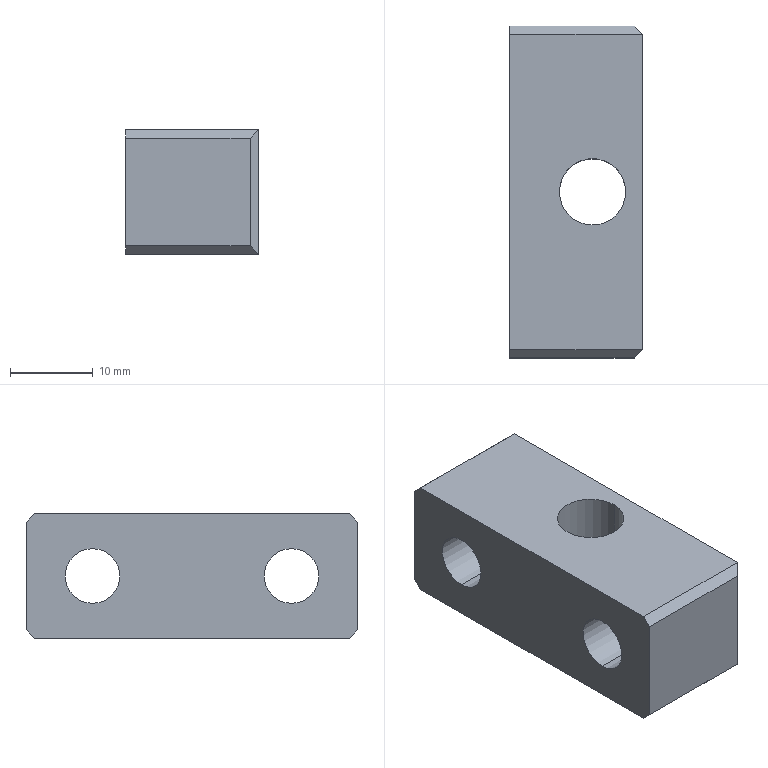Component | SolidWorks | ConveyorScrewAdjustmentSeat-2 | 1 solid | 24 faces | box 16 x 40 x 15 mm | volume 6635 mm3 | plane 14 | cylinder 10 | commonest cylinder face diameters 11 x4 6.6 x4 8 x2 | material Plain Carbon Steel
build123d program:
from build123d import *

# Parameters (mm, degrees)
SKETCH1_W                                            = 15
SKETCH1_H                                            = 40
BOSS_EXTRUDE1_DEPTH                                  = 16
HOLE_SIZE_ACCORDING_TO_TYPE_1_OF_HEXAGON_D           = 6.6
HOLE_SIZE_ACCORDING_TO_TYPE_1_OF_HEXAGON_CBORE_D     = 11
HOLE_SIZE_ACCORDING_TO_TYPE_1_OF_HEXAGON_CBORE_DEPTH = 8.8
M8_TAPPED_HOLE1_D                                    = 8
CHAMFER1_SIZE                                        = 1


with BuildPart() as part:
    # Sketch1 → Boss-Extrude1 (new body)
    with BuildSketch(Plane(origin=(0, 0, 0), x_dir=(0, 0, -1), z_dir=(1, 0, 0))):
        Rectangle(SKETCH1_W, SKETCH1_H)
    extrude(amount=BOSS_EXTRUDE1_DEPTH)

    # Hole Size according to type 1 of hexagon (through all)
    with Locations(Plane(origin=(16, 0, 0), x_dir=(0, 0, -1), z_dir=(1, 0, 0))):
        with Locations((0, 12), (0, -12)):
            CounterBoreHole(HOLE_SIZE_ACCORDING_TO_TYPE_1_OF_HEXAGON_D / 2, HOLE_SIZE_ACCORDING_TO_TYPE_1_OF_HEXAGON_CBORE_D / 2, HOLE_SIZE_ACCORDING_TO_TYPE_1_OF_HEXAGON_CBORE_DEPTH)

    # M8 Tapped Hole1 (through all)
    with Locations(Plane.XY.offset(7.5)):
        with Locations((10, 0)):
            Hole(M8_TAPPED_HOLE1_D / 2)

    # Chamfer1
    chamfer1_edges = [part.edges().sort_by_distance(p)[0] for p in [
        (16, -20, 0),
        (16, 20, 0),
        (8, -20, -7.5),
        (8, -20, 7.5),
        (8, 20, 7.5),
        (8, 20, -7.5),
    ]]
    chamfer(chamfer1_edges, length=CHAMFER1_SIZE)


solid = part.part

# Placed as in the assembly
solid = solid.moved(Location((47.45, 5.646, 262.5), (0, 0, 0)))
STEP:
#1=COLOUR_RGB('',0.7922,0.8196,0.9333);
#2=FILL_AREA_STYLE_COLOUR('',#1);
#3=FILL_AREA_STYLE('',(#2));
#4=SURFACE_STYLE_FILL_AREA(#3);
#5=SURFACE_SIDE_STYLE('',(#4));
#6=SURFACE_STYLE_USAGE(.BOTH.,#5);
#7=PRESENTATION_STYLE_ASSIGNMENT((#6));
#8=CARTESIAN_POINT('',(2.104,0.2223,10.039));
#9=VERTEX_POINT('',#8);
#10=CARTESIAN_POINT('',(2.419,0.2223,10.039));
#11=VERTEX_POINT('',#10);
#12=CARTESIAN_POINT('',(2.262,0.2223,10.039));
#13=DIRECTION('',(0.,0.,1.));
#14=DIRECTION('',(1.,0.,0.));
#15=AXIS2_PLACEMENT_3D('',#12,#13,#14);
#16=CIRCLE('',#15,0.1575);
#17=EDGE_CURVE('',#9,#11,#16,.T.);
#18=ORIENTED_EDGE('',*,*,#17,.F.);
#19=CARTESIAN_POINT('',(2.104,0.2223,10.63));
#20=VERTEX_POINT('',#19);
#21=CARTESIAN_POINT('',(2.104,0.2223,10.63));
#22=DIRECTION('',(0.,0.,1.));
#23=VECTOR('',#22,39.37);
#24=LINE('',#21,#23);
#25=EDGE_CURVE('',#9,#20,#24,.T.);
#26=ORIENTED_EDGE('',*,*,#25,.T.);
#27=CARTESIAN_POINT('',(2.419,0.2223,10.63));
#28=VERTEX_POINT('',#27);
#29=CARTESIAN_POINT('',(2.262,0.2223,10.63));
#30=DIRECTION('',(0.,0.,1.));
#31=DIRECTION('',(1.,0.,0.));
#32=AXIS2_PLACEMENT_3D('',#29,#30,#31);
#33=CIRCLE('',#32,0.1575);
#34=EDGE_CURVE('',#20,#28,#33,.T.);
#35=ORIENTED_EDGE('',*,*,#34,.T.);
#36=CARTESIAN_POINT('',(2.419,0.2223,10.63));
#37=DIRECTION('',(0.,0.,1.));
#38=VECTOR('',#37,39.37);
#39=LINE('',#36,#38);
#40=EDGE_CURVE('',#11,#28,#39,.T.);
#41=ORIENTED_EDGE('',*,*,#40,.F.);
#42=EDGE_LOOP('',(#18,#26,#35,#41));
#43=FACE_OUTER_BOUND('',#42,.T.);
#44=CARTESIAN_POINT('',(2.262,0.2223,10.63));
#45=DIRECTION('',(0.,0.,1.));
#46=DIRECTION('',(1.,0.,0.));
#47=AXIS2_PLACEMENT_3D('',#44,#45,#46);
#48=CYLINDRICAL_SURFACE('',#47,0.1575);
#49=ADVANCED_FACE('',(#43),#48,.F.);
#50=CARTESIAN_POINT('',(2.152,0.6947,10.551));
#51=VERTEX_POINT('',#50);
#52=CARTESIAN_POINT('',(2.152,0.6947,10.118));
#53=VERTEX_POINT('',#52);
#54=CARTESIAN_POINT('',(2.152,0.6947,10.335));
#55=DIRECTION('',(1.,0.,0.));
#56=DIRECTION('',(0.,0.,-1.));
#57=AXIS2_PLACEMENT_3D('',#54,#55,#56);
#58=CIRCLE('',#57,0.2165);
#59=EDGE_CURVE('',#51,#53,#58,.T.);
#60=ORIENTED_EDGE('',*,*,#59,.F.);
#61=CARTESIAN_POINT('',(2.498,0.6947,10.551));
#62=VERTEX_POINT('',#61);
#63=CARTESIAN_POINT('',(2.498,0.6947,10.551));
#64=DIRECTION('',(1.,0.,0.));
#65=VECTOR('',#64,39.37);
#66=LINE('',#63,#65);
#67=EDGE_CURVE('',#51,#62,#66,.T.);
#68=ORIENTED_EDGE('',*,*,#67,.T.);
#69=CARTESIAN_POINT('',(2.498,0.6947,10.118));
#70=VERTEX_POINT('',#69);
#71=CARTESIAN_POINT('',(2.498,0.6947,10.335));
#72=DIRECTION('',(1.,0.,0.));
#73=DIRECTION('',(0.,0.,-1.));
#74=AXIS2_PLACEMENT_3D('',#71,#72,#73);
#75=CIRCLE('',#74,0.2165);
#76=EDGE_CURVE('',#62,#70,#75,.T.);
#77=ORIENTED_EDGE('',*,*,#76,.T.);
#78=CARTESIAN_POINT('',(2.498,0.6947,10.118));
#79=DIRECTION('',(1.,0.,0.));
#80=VECTOR('',#79,39.37);
#81=LINE('',#78,#80);
#82=EDGE_CURVE('',#53,#70,#81,.T.);
#83=ORIENTED_EDGE('',*,*,#82,.F.);
#84=EDGE_LOOP('',(#60,#68,#77,#83));
#85=FACE_OUTER_BOUND('',#84,.T.);
#86=CARTESIAN_POINT('',(2.498,0.6947,10.335));
#87=DIRECTION('',(1.,0.,0.));
#88=DIRECTION('',(0.,0.,-1.));
#89=AXIS2_PLACEMENT_3D('',#86,#87,#88);
#90=CYLINDRICAL_SURFACE('',#89,0.2165);
#91=ADVANCED_FACE('',(#85),#90,.F.);
#92=CARTESIAN_POINT('',(1.868,0.6947,10.465));
#93=VERTEX_POINT('',#92);
#94=CARTESIAN_POINT('',(1.868,0.6947,10.205));
#95=VERTEX_POINT('',#94);
#96=CARTESIAN_POINT('',(1.868,0.6947,10.335));
#97=DIRECTION('',(1.,0.,0.));
#98=DIRECTION('',(0.,0.,-1.));
#99=AXIS2_PLACEMENT_3D('',#96,#97,#98);
#100=CIRCLE('',#99,0.1299);
#101=EDGE_CURVE('',#93,#95,#100,.T.);
#102=ORIENTED_EDGE('',*,*,#101,.F.);
#103=CARTESIAN_POINT('',(2.152,0.6947,10.465));
#104=VERTEX_POINT('',#103);
#105=CARTESIAN_POINT('',(2.498,0.6947,10.465));
#106=DIRECTION('',(1.,0.,0.));
#107=VECTOR('',#106,39.37);
#108=LINE('',#105,#107);
#109=EDGE_CURVE('',#93,#104,#108,.T.);
#110=ORIENTED_EDGE('',*,*,#109,.T.);
#111=CARTESIAN_POINT('',(2.152,0.6947,10.205));
#112=VERTEX_POINT('',#111);
#113=CARTESIAN_POINT('',(2.152,0.6947,10.335));
#114=DIRECTION('',(1.,0.,0.));
#115=DIRECTION('',(0.,0.,-1.));
#116=AXIS2_PLACEMENT_3D('',#113,#114,#115);
#117=CIRCLE('',#116,0.1299);
#118=EDGE_CURVE('',#104,#112,#117,.T.);
#119=ORIENTED_EDGE('',*,*,#118,.T.);
#120=CARTESIAN_POINT('',(2.498,0.6947,10.205));
#121=DIRECTION('',(1.,0.,0.));
#122=VECTOR('',#121,39.37);
#123=LINE('',#120,#122);
#124=EDGE_CURVE('',#95,#112,#123,.T.);
#125=ORIENTED_EDGE('',*,*,#124,.F.);
#126=EDGE_LOOP('',(#102,#110,#119,#125));
#127=FACE_OUTER_BOUND('',#126,.T.);
#128=CARTESIAN_POINT('',(2.498,0.6947,10.335));
#129=DIRECTION('',(1.,0.,0.));
#130=DIRECTION('',(0.,0.,-1.));
#131=AXIS2_PLACEMENT_3D('',#128,#129,#130);
#132=CYLINDRICAL_SURFACE('',#131,0.1299);
#133=ADVANCED_FACE('',(#127),#132,.F.);
#134=CARTESIAN_POINT('',(2.152,-0.2502,10.551));
#135=VERTEX_POINT('',#134);
#136=CARTESIAN_POINT('',(2.152,-0.2502,10.118));
#137=VERTEX_POINT('',#136);
#138=CARTESIAN_POINT('',(2.152,-0.2502,10.335));
#139=DIRECTION('',(1.,0.,0.));
#140=DIRECTION('',(0.,0.,-1.));
#141=AXIS2_PLACEMENT_3D('',#138,#139,#140);
#142=CIRCLE('',#141,0.2165);
#143=EDGE_CURVE('',#135,#137,#142,.T.);
#144=ORIENTED_EDGE('',*,*,#143,.F.);
#145=CARTESIAN_POINT('',(2.498,-0.2502,10.551));
#146=VERTEX_POINT('',#145);
#147=CARTESIAN_POINT('',(2.498,-0.2502,10.551));
#148=DIRECTION('',(1.,0.,0.));
#149=VECTOR('',#148,39.37);
#150=LINE('',#147,#149);
#151=EDGE_CURVE('',#135,#146,#150,.T.);
#152=ORIENTED_EDGE('',*,*,#151,.T.);
#153=CARTESIAN_POINT('',(2.498,-0.2502,10.118));
#154=VERTEX_POINT('',#153);
#155=CARTESIAN_POINT('',(2.498,-0.2502,10.335));
#156=DIRECTION('',(1.,0.,0.));
#157=DIRECTION('',(0.,0.,-1.));
#158=AXIS2_PLACEMENT_3D('',#155,#156,#157);
#159=CIRCLE('',#158,0.2165);
#160=EDGE_CURVE('',#146,#154,#159,.T.);
#161=ORIENTED_EDGE('',*,*,#160,.T.);
#162=CARTESIAN_POINT('',(2.498,-0.2502,10.118));
#163=DIRECTION('',(1.,0.,0.));
#164=VECTOR('',#163,39.37);
#165=LINE('',#162,#164);
#166=EDGE_CURVE('',#137,#154,#165,.T.);
#167=ORIENTED_EDGE('',*,*,#166,.F.);
#168=EDGE_LOOP('',(#144,#152,#161,#167));
#169=FACE_OUTER_BOUND('',#168,.T.);
#170=CARTESIAN_POINT('',(2.498,-0.2502,10.335));
#171=DIRECTION('',(1.,0.,0.));
#172=DIRECTION('',(0.,0.,-1.));
#173=AXIS2_PLACEMENT_3D('',#170,#171,#172);
#174=CYLINDRICAL_SURFACE('',#173,0.2165);
#175=ADVANCED_FACE('',(#169),#174,.F.);
#176=CARTESIAN_POINT('',(1.868,-0.2502,10.465));
#177=VERTEX_POINT('',#176);
#178=CARTESIAN_POINT('',(1.868,-0.2502,10.205));
#179=VERTEX_POINT('',#178);
#180=CARTESIAN_POINT('',(1.868,-0.2502,10.335));
#181=DIRECTION('',(1.,0.,0.));
#182=DIRECTION('',(0.,0.,-1.));
#183=AXIS2_PLACEMENT_3D('',#180,#181,#182);
#184=CIRCLE('',#183,0.1299);
#185=EDGE_CURVE('',#177,#179,#184,.T.);
#186=ORIENTED_EDGE('',*,*,#185,.F.);
#187=CARTESIAN_POINT('',(2.152,-0.2502,10.465));
#188=VERTEX_POINT('',#187);
#189=CARTESIAN_POINT('',(2.498,-0.2502,10.465));
#190=DIRECTION('',(1.,0.,0.));
#191=VECTOR('',#190,39.37);
#192=LINE('',#189,#191);
#193=EDGE_CURVE('',#177,#188,#192,.T.);
#194=ORIENTED_EDGE('',*,*,#193,.T.);
#195=CARTESIAN_POINT('',(2.152,-0.2502,10.205));
#196=VERTEX_POINT('',#195);
#197=CARTESIAN_POINT('',(2.152,-0.2502,10.335));
#198=DIRECTION('',(1.,0.,0.));
#199=DIRECTION('',(0.,0.,-1.));
#200=AXIS2_PLACEMENT_3D('',#197,#198,#199);
#201=CIRCLE('',#200,0.1299);
#202=EDGE_CURVE('',#188,#196,#201,.T.);
#203=ORIENTED_EDGE('',*,*,#202,.T.);
#204=CARTESIAN_POINT('',(2.498,-0.2502,10.205));
#205=DIRECTION('',(1.,0.,0.));
#206=VECTOR('',#205,39.37);
#207=LINE('',#204,#206);
#208=EDGE_CURVE('',#179,#196,#207,.T.);
#209=ORIENTED_EDGE('',*,*,#208,.F.);
#210=EDGE_LOOP('',(#186,#194,#203,#209));
#211=FACE_OUTER_BOUND('',#210,.T.);
#212=CARTESIAN_POINT('',(2.498,-0.2502,10.335));
#213=DIRECTION('',(1.,0.,0.));
#214=DIRECTION('',(0.,0.,-1.));
#215=AXIS2_PLACEMENT_3D('',#212,#213,#214);
#216=CYLINDRICAL_SURFACE('',#215,0.1299);
#217=ADVANCED_FACE('',(#211),#216,.F.);
#218=CARTESIAN_POINT('',(2.262,0.2223,10.039));
#219=DIRECTION('',(0.,0.,1.));
#220=DIRECTION('',(1.,0.,0.));
#221=AXIS2_PLACEMENT_3D('',#218,#219,#220);
#222=CIRCLE('',#221,0.1575);
#223=EDGE_CURVE('',#11,#9,#222,.T.);
#224=ORIENTED_EDGE('',*,*,#223,.T.);
#225=ORIENTED_EDGE('',*,*,#17,.T.);
#226=EDGE_LOOP('',(#224,#225));
#227=FACE_BOUND('',#226,.T.);
#228=CARTESIAN_POINT('',(2.498,-0.5258,10.039));
#229=VERTEX_POINT('',#228);
#230=CARTESIAN_POINT('',(2.498,0.9703,10.039));
#231=VERTEX_POINT('',#230);
#232=CARTESIAN_POINT('',(2.498,-0.5651,10.039));
#233=DIRECTION('',(0.,1.,0.));
#234=VECTOR('',#233,39.37);
#235=LINE('',#232,#234);
#236=EDGE_CURVE('',#229,#231,#235,.T.);
#237=ORIENTED_EDGE('',*,*,#236,.F.);
#238=CARTESIAN_POINT('',(1.868,-0.5258,10.039));
#239=VERTEX_POINT('',#238);
#240=CARTESIAN_POINT('',(2.498,-0.5258,10.039));
#241=DIRECTION('',(-1.,0.,0.));
#242=VECTOR('',#241,39.37);
#243=LINE('',#240,#242);
#244=EDGE_CURVE('',#229,#239,#243,.T.);
#245=ORIENTED_EDGE('',*,*,#244,.T.);
#246=CARTESIAN_POINT('',(1.868,0.9703,10.039));
#247=VERTEX_POINT('',#246);
#248=CARTESIAN_POINT('',(1.868,-0.5651,10.039));
#249=DIRECTION('',(0.,1.,0.));
#250=VECTOR('',#249,39.37);
#251=LINE('',#248,#250);
#252=EDGE_CURVE('',#239,#247,#251,.T.);
#253=ORIENTED_EDGE('',*,*,#252,.T.);
#254=CARTESIAN_POINT('',(2.498,0.9703,10.039));
#255=DIRECTION('',(1.,0.,0.));
#256=VECTOR('',#255,39.37);
#257=LINE('',#254,#256);
#258=EDGE_CURVE('',#247,#231,#257,.T.);
#259=ORIENTED_EDGE('',*,*,#258,.T.);
#260=EDGE_LOOP('',(#237,#245,#253,#259));
#261=FACE_OUTER_BOUND('',#260,.T.);
#262=CARTESIAN_POINT('',(2.498,-0.5651,10.039));
#263=DIRECTION('',(0.,0.,1.));
#264=DIRECTION('',(1.,0.,0.));
#265=AXIS2_PLACEMENT_3D('',#262,#263,#264);
#266=PLANE('',#265);
#267=ADVANCED_FACE('',(#227,#261),#266,.F.);
#268=CARTESIAN_POINT('',(1.868,1.01,10.079));
#269=VERTEX_POINT('',#268);
#270=CARTESIAN_POINT('',(1.868,1.01,10.591));
#271=VERTEX_POINT('',#270);
#272=CARTESIAN_POINT('',(1.868,1.01,10.63));
#273=DIRECTION('',(0.,0.,1.));
#274=VECTOR('',#273,39.37);
#275=LINE('',#272,#274);
#276=EDGE_CURVE('',#269,#271,#275,.T.);
#277=ORIENTED_EDGE('',*,*,#276,.T.);
#278=CARTESIAN_POINT('',(2.459,1.01,10.591));
#279=VERTEX_POINT('',#278);
#280=CARTESIAN_POINT('',(2.498,1.01,10.591));
#281=DIRECTION('',(1.,0.,0.));
#282=VECTOR('',#281,39.37);
#283=LINE('',#280,#282);
#284=EDGE_CURVE('',#271,#279,#283,.T.);
#285=ORIENTED_EDGE('',*,*,#284,.T.);
#286=CARTESIAN_POINT('',(2.459,1.01,10.079));
#287=VERTEX_POINT('',#286);
#288=CARTESIAN_POINT('',(2.459,1.01,10.63));
#289=DIRECTION('',(0.,0.,-1.));
#290=VECTOR('',#289,39.37);
#291=LINE('',#288,#290);
#292=EDGE_CURVE('',#279,#287,#291,.T.);
#293=ORIENTED_EDGE('',*,*,#292,.T.);
#294=CARTESIAN_POINT('',(2.498,1.01,10.079));
#295=DIRECTION('',(-1.,0.,0.));
#296=VECTOR('',#295,39.37);
#297=LINE('',#294,#296);
#298=EDGE_CURVE('',#287,#269,#297,.T.);
#299=ORIENTED_EDGE('',*,*,#298,.T.);
#300=EDGE_LOOP('',(#277,#285,#293,#299));
#301=FACE_OUTER_BOUND('',#300,.T.);
#302=CARTESIAN_POINT('',(2.498,1.01,10.63));
#303=DIRECTION('',(0.,-1.,0.));
#304=DIRECTION('',(0.,0.,-1.));
#305=AXIS2_PLACEMENT_3D('',#302,#303,#304);
#306=PLANE('',#305);
#307=ADVANCED_FACE('',(#301),#306,.F.);
#308=CARTESIAN_POINT('',(2.262,0.2223,10.63));
#309=DIRECTION('',(0.,0.,1.));
#310=DIRECTION('',(1.,0.,0.));
#311=AXIS2_PLACEMENT_3D('',#308,#309,#310);
#312=CIRCLE('',#311,0.1575);
#313=EDGE_CURVE('',#28,#20,#312,.T.);
#314=ORIENTED_EDGE('',*,*,#313,.F.);
#315=ORIENTED_EDGE('',*,*,#34,.F.);
#316=EDGE_LOOP('',(#314,#315));
#317=FACE_BOUND('',#316,.T.);
#318=CARTESIAN_POINT('',(1.868,0.9703,10.63));
#319=VERTEX_POINT('',#318);
#320=CARTESIAN_POINT('',(1.868,-0.5258,10.63));
#321=VERTEX_POINT('',#320);
#322=CARTESIAN_POINT('',(1.868,-0.5651,10.63));
#323=DIRECTION('',(0.,-1.,0.));
#324=VECTOR('',#323,39.37);
#325=LINE('',#322,#324);
#326=EDGE_CURVE('',#319,#321,#325,.T.);
#327=ORIENTED_EDGE('',*,*,#326,.T.);
#328=CARTESIAN_POINT('',(2.498,-0.5258,10.63));
#329=VERTEX_POINT('',#328);
#330=CARTESIAN_POINT('',(2.498,-0.5258,10.63));
#331=DIRECTION('',(1.,0.,0.));
#332=VECTOR('',#331,39.37);
#333=LINE('',#330,#332);
#334=EDGE_CURVE('',#321,#329,#333,.T.);
#335=ORIENTED_EDGE('',*,*,#334,.T.);
#336=CARTESIAN_POINT('',(2.498,0.9703,10.63));
#337=VERTEX_POINT('',#336);
#338=CARTESIAN_POINT('',(2.498,-0.5651,10.63));
#339=DIRECTION('',(0.,-1.,0.));
#340=VECTOR('',#339,39.37);
#341=LINE('',#338,#340);
#342=EDGE_CURVE('',#337,#329,#341,.T.);
#343=ORIENTED_EDGE('',*,*,#342,.F.);
#344=CARTESIAN_POINT('',(2.498,0.9703,10.63));
#345=DIRECTION('',(-1.,0.,0.));
#346=VECTOR('',#345,39.37);
#347=LINE('',#344,#346);
#348=EDGE_CURVE('',#337,#319,#347,.T.);
#349=ORIENTED_EDGE('',*,*,#348,.T.);
#350=EDGE_LOOP('',(#327,#335,#343,#349));
#351=FACE_OUTER_BOUND('',#350,.T.);
#352=CARTESIAN_POINT('',(2.498,-0.5651,10.63));
#353=DIRECTION('',(0.,0.,-1.));
#354=DIRECTION('',(-1.,0.,0.));
#355=AXIS2_PLACEMENT_3D('',#352,#353,#354);
#356=PLANE('',#355);
#357=ADVANCED_FACE('',(#317,#351),#356,.F.);
#358=CARTESIAN_POINT('',(1.868,-0.5651,10.591));
#359=VERTEX_POINT('',#358);
#360=CARTESIAN_POINT('',(1.868,-0.5651,10.079));
#361=VERTEX_POINT('',#360);
#362=CARTESIAN_POINT('',(1.868,-0.5651,10.63));
#363=DIRECTION('',(0.,0.,-1.));
#364=VECTOR('',#363,39.37);
#365=LINE('',#362,#364);
#366=EDGE_CURVE('',#359,#361,#365,.T.);
#367=ORIENTED_EDGE('',*,*,#366,.T.);
#368=CARTESIAN_POINT('',(2.459,-0.5651,10.079));
#369=VERTEX_POINT('',#368);
#370=CARTESIAN_POINT('',(2.498,-0.5651,10.079));
#371=DIRECTION('',(1.,0.,0.));
#372=VECTOR('',#371,39.37);
#373=LINE('',#370,#372);
#374=EDGE_CURVE('',#361,#369,#373,.T.);
#375=ORIENTED_EDGE('',*,*,#374,.T.);
#376=CARTESIAN_POINT('',(2.459,-0.5651,10.591));
#377=VERTEX_POINT('',#376);
#378=CARTESIAN_POINT('',(2.459,-0.5651,10.63));
#379=DIRECTION('',(0.,0.,1.));
#380=VECTOR('',#379,39.37);
#381=LINE('',#378,#380);
#382=EDGE_CURVE('',#369,#377,#381,.T.);
#383=ORIENTED_EDGE('',*,*,#382,.T.);
#384=CARTESIAN_POINT('',(2.498,-0.5651,10.591));
#385=DIRECTION('',(-1.,0.,0.));
#386=VECTOR('',#385,39.37);
#387=LINE('',#384,#386);
#388=EDGE_CURVE('',#377,#359,#387,.T.);
#389=ORIENTED_EDGE('',*,*,#388,.T.);
#390=EDGE_LOOP('',(#367,#375,#383,#389));
#391=FACE_OUTER_BOUND('',#390,.T.);
#392=CARTESIAN_POINT('',(2.498,-0.5651,10.63));
#393=DIRECTION('',(0.,1.,0.));
#394=DIRECTION('',(0.,0.,1.));
#395=AXIS2_PLACEMENT_3D('',#392,#393,#394);
#396=PLANE('',#395);
#397=ADVANCED_FACE('',(#391),#396,.F.);
#398=CARTESIAN_POINT('',(2.498,0.6947,10.335));
#399=DIRECTION('',(1.,0.,0.));
#400=DIRECTION('',(0.,0.,-1.));
#401=AXIS2_PLACEMENT_3D('',#398,#399,#400);
#402=CIRCLE('',#401,0.2165);
#403=EDGE_CURVE('',#70,#62,#402,.T.);
#404=ORIENTED_EDGE('',*,*,#403,.F.);
#405=ORIENTED_EDGE('',*,*,#76,.F.);
#406=EDGE_LOOP('',(#404,#405));
#407=FACE_BOUND('',#406,.T.);
#408=CARTESIAN_POINT('',(2.498,-0.2502,10.335));
#409=DIRECTION('',(1.,0.,0.));
#410=DIRECTION('',(0.,0.,-1.));
#411=AXIS2_PLACEMENT_3D('',#408,#409,#410);
#412=CIRCLE('',#411,0.2165);
#413=EDGE_CURVE('',#154,#146,#412,.T.);
#414=ORIENTED_EDGE('',*,*,#413,.F.);
#415=ORIENTED_EDGE('',*,*,#160,.F.);
#416=EDGE_LOOP('',(#414,#415));
#417=FACE_BOUND('',#416,.T.);
#418=ORIENTED_EDGE('',*,*,#342,.T.);
#419=CARTESIAN_POINT('',(2.498,-0.5258,10.335));
#420=DIRECTION('',(0.,0.,-1.));
#421=VECTOR('',#420,39.37);
#422=LINE('',#419,#421);
#423=EDGE_CURVE('',#329,#229,#422,.T.);
#424=ORIENTED_EDGE('',*,*,#423,.T.);
#425=ORIENTED_EDGE('',*,*,#236,.T.);
#426=CARTESIAN_POINT('',(2.498,0.9703,10.335));
#427=DIRECTION('',(0.,0.,1.));
#428=VECTOR('',#427,39.37);
#429=LINE('',#426,#428);
#430=EDGE_CURVE('',#231,#337,#429,.T.);
#431=ORIENTED_EDGE('',*,*,#430,.T.);
#432=EDGE_LOOP('',(#418,#424,#425,#431));
#433=FACE_OUTER_BOUND('',#432,.T.);
#434=CARTESIAN_POINT('',(2.498,0.2223,10.335));
#435=DIRECTION('',(-1.,0.,0.));
#436=DIRECTION('',(0.,0.,1.));
#437=AXIS2_PLACEMENT_3D('',#434,#435,#436);
#438=PLANE('',#437);
#439=ADVANCED_FACE('',(#407,#417,#433),#438,.F.);
#440=CARTESIAN_POINT('',(1.868,0.6947,10.335));
#441=DIRECTION('',(1.,0.,0.));
#442=DIRECTION('',(0.,0.,-1.));
#443=AXIS2_PLACEMENT_3D('',#440,#441,#442);
#444=CIRCLE('',#443,0.1299);
#445=EDGE_CURVE('',#95,#93,#444,.T.);
#446=ORIENTED_EDGE('',*,*,#445,.T.);
#447=ORIENTED_EDGE('',*,*,#101,.T.);
#448=EDGE_LOOP('',(#446,#447));
#449=FACE_BOUND('',#448,.T.);
#450=CARTESIAN_POINT('',(1.868,-0.2502,10.335));
#451=DIRECTION('',(1.,0.,0.));
#452=DIRECTION('',(0.,0.,-1.));
#453=AXIS2_PLACEMENT_3D('',#450,#451,#452);
#454=CIRCLE('',#453,0.1299);
#455=EDGE_CURVE('',#179,#177,#454,.T.);
#456=ORIENTED_EDGE('',*,*,#455,.T.);
#457=ORIENTED_EDGE('',*,*,#185,.T.);
#458=EDGE_LOOP('',(#456,#457));
#459=FACE_BOUND('',#458,.T.);
#460=ORIENTED_EDGE('',*,*,#252,.F.);
#461=CARTESIAN_POINT('',(1.868,-0.2994,9.813));
#462=DIRECTION('',(0.,-0.7071,0.7071));
#463=VECTOR('',#462,39.37);
#464=LINE('',#461,#463);
#465=EDGE_CURVE('',#239,#361,#464,.T.);
#466=ORIENTED_EDGE('',*,*,#465,.T.);
#467=ORIENTED_EDGE('',*,*,#366,.F.);
#468=CARTESIAN_POINT('',(1.868,-0.2994,10.856));
#469=DIRECTION('',(0.,0.7071,0.7071));
#470=VECTOR('',#469,39.37);
#471=LINE('',#468,#470);
#472=EDGE_CURVE('',#359,#321,#471,.T.);
#473=ORIENTED_EDGE('',*,*,#472,.T.);
#474=ORIENTED_EDGE('',*,*,#326,.F.);
#475=CARTESIAN_POINT('',(1.868,0.7439,10.856));
#476=DIRECTION('',(0.,0.7071,-0.7071));
#477=VECTOR('',#476,39.37);
#478=LINE('',#475,#477);
#479=EDGE_CURVE('',#319,#271,#478,.T.);
#480=ORIENTED_EDGE('',*,*,#479,.T.);
#481=ORIENTED_EDGE('',*,*,#276,.F.);
#482=CARTESIAN_POINT('',(1.868,0.7439,9.813));
#483=DIRECTION('',(0.,-0.7071,-0.7071));
#484=VECTOR('',#483,39.37);
#485=LINE('',#482,#484);
#486=EDGE_CURVE('',#269,#247,#485,.T.);
#487=ORIENTED_EDGE('',*,*,#486,.T.);
#488=EDGE_LOOP('',(#460,#466,#467,#473,#474,#480,#481,#487));
#489=FACE_OUTER_BOUND('',#488,.T.);
#490=CARTESIAN_POINT('',(1.868,0.2223,10.335));
#491=DIRECTION('',(-1.,0.,0.));
#492=DIRECTION('',(0.,0.,1.));
#493=AXIS2_PLACEMENT_3D('',#490,#491,#492);
#494=PLANE('',#493);
#495=ADVANCED_FACE('',(#449,#459,#489),#494,.T.);
#496=ORIENTED_EDGE('',*,*,#193,.F.);
#497=ORIENTED_EDGE('',*,*,#455,.F.);
#498=ORIENTED_EDGE('',*,*,#208,.T.);
#499=CARTESIAN_POINT('',(2.152,-0.2502,10.335));
#500=DIRECTION('',(1.,0.,0.));
#501=DIRECTION('',(0.,0.,-1.));
#502=AXIS2_PLACEMENT_3D('',#499,#500,#501);
#503=CIRCLE('',#502,0.1299);
#504=EDGE_CURVE('',#196,#188,#503,.T.);
#505=ORIENTED_EDGE('',*,*,#504,.T.);
#506=EDGE_LOOP('',(#496,#497,#498,#505));
#507=FACE_OUTER_BOUND('',#506,.T.);
#508=CARTESIAN_POINT('',(2.498,-0.2502,10.335));
#509=DIRECTION('',(1.,0.,0.));
#510=DIRECTION('',(0.,0.,-1.));
#511=AXIS2_PLACEMENT_3D('',#508,#509,#510);
#512=CYLINDRICAL_SURFACE('',#511,0.1299);
#513=ADVANCED_FACE('',(#507),#512,.F.);
#514=ORIENTED_EDGE('',*,*,#504,.F.);
#515=ORIENTED_EDGE('',*,*,#202,.F.);
#516=EDGE_LOOP('',(#514,#515));
#517=FACE_BOUND('',#516,.T.);
#518=CARTESIAN_POINT('',(2.152,-0.2502,10.335));
#519=DIRECTION('',(1.,0.,0.));
#520=DIRECTION('',(0.,0.,-1.));
#521=AXIS2_PLACEMENT_3D('',#518,#519,#520);
#522=CIRCLE('',#521,0.2165);
#523=EDGE_CURVE('',#137,#135,#522,.T.);
#524=ORIENTED_EDGE('',*,*,#523,.T.);
#525=ORIENTED_EDGE('',*,*,#143,.T.);
#526=EDGE_LOOP('',(#524,#525));
#527=FACE_OUTER_BOUND('',#526,.T.);
#528=CARTESIAN_POINT('',(2.152,-0.1202,10.335));
#529=DIRECTION('',(-1.,0.,0.));
#530=DIRECTION('',(0.,0.,1.));
#531=AXIS2_PLACEMENT_3D('',#528,#529,#530);
#532=PLANE('',#531);
#533=ADVANCED_FACE('',(#517,#527),#532,.F.);
#534=ORIENTED_EDGE('',*,*,#151,.F.);
#535=ORIENTED_EDGE('',*,*,#523,.F.);
#536=ORIENTED_EDGE('',*,*,#166,.T.);
#537=ORIENTED_EDGE('',*,*,#413,.T.);
#538=EDGE_LOOP('',(#534,#535,#536,#537));
#539=FACE_OUTER_BOUND('',#538,.T.);
#540=CARTESIAN_POINT('',(2.498,-0.2502,10.335));
#541=DIRECTION('',(1.,0.,0.));
#542=DIRECTION('',(0.,0.,-1.));
#543=AXIS2_PLACEMENT_3D('',#540,#541,#542);
#544=CYLINDRICAL_SURFACE('',#543,0.2165);
#545=ADVANCED_FACE('',(#539),#544,.F.);
#546=ORIENTED_EDGE('',*,*,#109,.F.);
#547=ORIENTED_EDGE('',*,*,#445,.F.);
#548=ORIENTED_EDGE('',*,*,#124,.T.);
#549=CARTESIAN_POINT('',(2.152,0.6947,10.335));
#550=DIRECTION('',(1.,0.,0.));
#551=DIRECTION('',(0.,0.,-1.));
#552=AXIS2_PLACEMENT_3D('',#549,#550,#551);
#553=CIRCLE('',#552,0.1299);
#554=EDGE_CURVE('',#112,#104,#553,.T.);
#555=ORIENTED_EDGE('',*,*,#554,.T.);
#556=EDGE_LOOP('',(#546,#547,#548,#555));
#557=FACE_OUTER_BOUND('',#556,.T.);
#558=CARTESIAN_POINT('',(2.498,0.6947,10.335));
#559=DIRECTION('',(1.,0.,0.));
#560=DIRECTION('',(0.,0.,-1.));
#561=AXIS2_PLACEMENT_3D('',#558,#559,#560);
#562=CYLINDRICAL_SURFACE('',#561,0.1299);
#563=ADVANCED_FACE('',(#557),#562,.F.);
#564=ORIENTED_EDGE('',*,*,#554,.F.);
#565=ORIENTED_EDGE('',*,*,#118,.F.);
#566=EDGE_LOOP('',(#564,#565));
#567=FACE_BOUND('',#566,.T.);
#568=CARTESIAN_POINT('',(2.152,0.6947,10.335));
#569=DIRECTION('',(1.,0.,0.));
#570=DIRECTION('',(0.,0.,-1.));
#571=AXIS2_PLACEMENT_3D('',#568,#569,#570);
#572=CIRCLE('',#571,0.2165);
#573=EDGE_CURVE('',#53,#51,#572,.T.);
#574=ORIENTED_EDGE('',*,*,#573,.T.);
#575=ORIENTED_EDGE('',*,*,#59,.T.);
#576=EDGE_LOOP('',(#574,#575));
#577=FACE_OUTER_BOUND('',#576,.T.);
#578=CARTESIAN_POINT('',(2.152,0.8246,10.335));
#579=DIRECTION('',(-1.,0.,0.));
#580=DIRECTION('',(0.,0.,1.));
#581=AXIS2_PLACEMENT_3D('',#578,#579,#580);
#582=PLANE('',#581);
#583=ADVANCED_FACE('',(#567,#577),#582,.F.);
#584=ORIENTED_EDGE('',*,*,#67,.F.);
#585=ORIENTED_EDGE('',*,*,#573,.F.);
#586=ORIENTED_EDGE('',*,*,#82,.T.);
#587=ORIENTED_EDGE('',*,*,#403,.T.);
#588=EDGE_LOOP('',(#584,#585,#586,#587));
#589=FACE_OUTER_BOUND('',#588,.T.);
#590=CARTESIAN_POINT('',(2.498,0.6947,10.335));
#591=DIRECTION('',(1.,0.,0.));
#592=DIRECTION('',(0.,0.,-1.));
#593=AXIS2_PLACEMENT_3D('',#590,#591,#592);
#594=CYLINDRICAL_SURFACE('',#593,0.2165);
#595=ADVANCED_FACE('',(#589),#594,.F.);
#596=ORIENTED_EDGE('',*,*,#25,.F.);
#597=ORIENTED_EDGE('',*,*,#223,.F.);
#598=ORIENTED_EDGE('',*,*,#40,.T.);
#599=ORIENTED_EDGE('',*,*,#313,.T.);
#600=EDGE_LOOP('',(#596,#597,#598,#599));
#601=FACE_OUTER_BOUND('',#600,.T.);
#602=CARTESIAN_POINT('',(2.262,0.2223,10.63));
#603=DIRECTION('',(0.,0.,1.));
#604=DIRECTION('',(1.,0.,0.));
#605=AXIS2_PLACEMENT_3D('',#602,#603,#604);
#606=CYLINDRICAL_SURFACE('',#605,0.1575);
#607=ADVANCED_FACE('',(#601),#606,.F.);
#608=ORIENTED_EDGE('',*,*,#472,.F.);
#609=ORIENTED_EDGE('',*,*,#388,.F.);
#610=CARTESIAN_POINT('',(2.4,-0.6242,10.531));
#611=DIRECTION('',(-0.5774,-0.5774,-0.5774));
#612=VECTOR('',#611,39.37);
#613=LINE('',#610,#612);
#614=EDGE_CURVE('',#329,#377,#613,.T.);
#615=ORIENTED_EDGE('',*,*,#614,.F.);
#616=ORIENTED_EDGE('',*,*,#334,.F.);
#617=EDGE_LOOP('',(#608,#609,#615,#616));
#618=FACE_OUTER_BOUND('',#617,.T.);
#619=CARTESIAN_POINT('',(2.498,-0.5651,10.591));
#620=DIRECTION('',(0.,0.7071,-0.7071));
#621=DIRECTION('',(-1.,0.,0.));
#622=AXIS2_PLACEMENT_3D('',#619,#620,#621);
#623=PLANE('',#622);
#624=ADVANCED_FACE('',(#618),#623,.F.);
#625=ORIENTED_EDGE('',*,*,#614,.T.);
#626=ORIENTED_EDGE('',*,*,#382,.F.);
#627=CARTESIAN_POINT('',(2.4,-0.6242,10.138));
#628=DIRECTION('',(-0.5774,-0.5774,0.5774));
#629=VECTOR('',#628,39.37);
#630=LINE('',#627,#629);
#631=EDGE_CURVE('',#229,#369,#630,.T.);
#632=ORIENTED_EDGE('',*,*,#631,.F.);
#633=ORIENTED_EDGE('',*,*,#423,.F.);
#634=EDGE_LOOP('',(#625,#626,#632,#633));
#635=FACE_OUTER_BOUND('',#634,.T.);
#636=CARTESIAN_POINT('',(2.498,-0.5258,10.335));
#637=DIRECTION('',(-0.7071,0.7071,0.));
#638=DIRECTION('',(0.,0.,-1.));
#639=AXIS2_PLACEMENT_3D('',#636,#637,#638);
#640=PLANE('',#639);
#641=ADVANCED_FACE('',(#635),#640,.F.);
#642=ORIENTED_EDGE('',*,*,#631,.T.);
#643=ORIENTED_EDGE('',*,*,#374,.F.);
#644=ORIENTED_EDGE('',*,*,#465,.F.);
#645=ORIENTED_EDGE('',*,*,#244,.F.);
#646=EDGE_LOOP('',(#642,#643,#644,#645));
#647=FACE_OUTER_BOUND('',#646,.T.);
#648=CARTESIAN_POINT('',(2.498,-0.5258,10.039));
#649=DIRECTION('',(0.,0.7071,0.7071));
#650=DIRECTION('',(-1.,0.,0.));
#651=AXIS2_PLACEMENT_3D('',#648,#649,#650);
#652=PLANE('',#651);
#653=ADVANCED_FACE('',(#647),#652,.F.);
#654=ORIENTED_EDGE('',*,*,#486,.F.);
#655=ORIENTED_EDGE('',*,*,#298,.F.);
#656=CARTESIAN_POINT('',(2.4,1.069,10.138));
#657=DIRECTION('',(-0.5774,0.5774,0.5774));
#658=VECTOR('',#657,39.37);
#659=LINE('',#656,#658);
#660=EDGE_CURVE('',#231,#287,#659,.T.);
#661=ORIENTED_EDGE('',*,*,#660,.F.);
#662=ORIENTED_EDGE('',*,*,#258,.F.);
#663=EDGE_LOOP('',(#654,#655,#661,#662));
#664=FACE_OUTER_BOUND('',#663,.T.);
#665=CARTESIAN_POINT('',(2.498,1.01,10.079));
#666=DIRECTION('',(0.,-0.7071,0.7071));
#667=DIRECTION('',(-1.,0.,0.));
#668=AXIS2_PLACEMENT_3D('',#665,#666,#667);
#669=PLANE('',#668);
#670=ADVANCED_FACE('',(#664),#669,.F.);
#671=ORIENTED_EDGE('',*,*,#660,.T.);
#672=ORIENTED_EDGE('',*,*,#292,.F.);
#673=CARTESIAN_POINT('',(2.4,1.069,10.531));
#674=DIRECTION('',(-0.5774,0.5774,-0.5774));
#675=VECTOR('',#674,39.37);
#676=LINE('',#673,#675);
#677=EDGE_CURVE('',#337,#279,#676,.T.);
#678=ORIENTED_EDGE('',*,*,#677,.F.);
#679=ORIENTED_EDGE('',*,*,#430,.F.);
#680=EDGE_LOOP('',(#671,#672,#678,#679));
#681=FACE_OUTER_BOUND('',#680,.T.);
#682=CARTESIAN_POINT('',(2.498,0.9703,10.335));
#683=DIRECTION('',(-0.7071,-0.7071,0.));
#684=DIRECTION('',(0.,0.,1.));
#685=AXIS2_PLACEMENT_3D('',#682,#683,#684);
#686=PLANE('',#685);
#687=ADVANCED_FACE('',(#681),#686,.F.);
#688=ORIENTED_EDGE('',*,*,#677,.T.);
#689=ORIENTED_EDGE('',*,*,#284,.F.);
#690=ORIENTED_EDGE('',*,*,#479,.F.);
#691=ORIENTED_EDGE('',*,*,#348,.F.);
#692=EDGE_LOOP('',(#688,#689,#690,#691));
#693=FACE_OUTER_BOUND('',#692,.T.);
#694=CARTESIAN_POINT('',(2.498,0.9703,10.63));
#695=DIRECTION('',(0.,-0.7071,-0.7071));
#696=DIRECTION('',(-1.,0.,0.));
#697=AXIS2_PLACEMENT_3D('',#694,#695,#696);
#698=PLANE('',#697);
#699=ADVANCED_FACE('',(#693),#698,.F.);
#700=CLOSED_SHELL('',(#49,#91,#133,#175,#217,#267,#307,#357,#397,#439,#495,#513,#533,#545,#563,#583,#595,#607,#624,#641,#653,#670,#687,#699));
#701=MANIFOLD_SOLID_BREP('',#700);
#702=STYLED_ITEM('',(#7),#701);
#703=PRESENTATION_LAYER_ASSIGNMENT('','',(#702));
#704=CARTESIAN_POINT('',(0.,0.,0.));
#705=DIRECTION('',(0.,0.,1.));
#706=DIRECTION('',(1.,0.,0.));
#707=AXIS2_PLACEMENT_3D('',#704,#705,#706);
#708=(LENGTH_UNIT()NAMED_UNIT(*)SI_UNIT($,.METRE.));
#709=LENGTH_MEASURE_WITH_UNIT(LENGTH_MEASURE(0.0254),#708);
#710=DIMENSIONAL_EXPONENTS(1.,0.,0.,0.,0.,0.,0.);
#711=(CONVERSION_BASED_UNIT('',#709)LENGTH_UNIT()NAMED_UNIT(#710));
#712=UNCERTAINTY_MEASURE_WITH_UNIT(LENGTH_MEASURE(0.00001),#711,'','');
#713=(NAMED_UNIT(*)PLANE_ANGLE_UNIT()SI_UNIT($,.RADIAN.));
#714=(NAMED_UNIT(*)SI_UNIT($,.STERADIAN.)SOLID_ANGLE_UNIT());
#715=(GEOMETRIC_REPRESENTATION_CONTEXT(3)GLOBAL_UNCERTAINTY_ASSIGNED_CONTEXT((#712))GLOBAL_UNIT_ASSIGNED_CONTEXT((#711,#713,#714))REPRESENTATION_CONTEXT('',''));
#716=ADVANCED_BREP_SHAPE_REPRESENTATION('',(#701,#707),#715);
#717=(LENGTH_UNIT()NAMED_UNIT(*)SI_UNIT($,.METRE.));
#718=LENGTH_MEASURE_WITH_UNIT(LENGTH_MEASURE(0.0254),#717);
#719=DIMENSIONAL_EXPONENTS(1.,0.,0.,0.,0.,0.,0.);
#720=(CONVERSION_BASED_UNIT('',#718)LENGTH_UNIT()NAMED_UNIT(#719));
#721=UNCERTAINTY_MEASURE_WITH_UNIT(LENGTH_MEASURE(0.00001),#720,'','');
#722=(NAMED_UNIT(*)PLANE_ANGLE_UNIT()SI_UNIT($,.RADIAN.));
#723=(NAMED_UNIT(*)SI_UNIT($,.STERADIAN.)SOLID_ANGLE_UNIT());
#724=(GEOMETRIC_REPRESENTATION_CONTEXT(3)GLOBAL_UNCERTAINTY_ASSIGNED_CONTEXT((#721))GLOBAL_UNIT_ASSIGNED_CONTEXT((#720,#722,#723))REPRESENTATION_CONTEXT('',''));
#725=MECHANICAL_DESIGN_GEOMETRIC_PRESENTATION_REPRESENTATION('',(#702),#724);